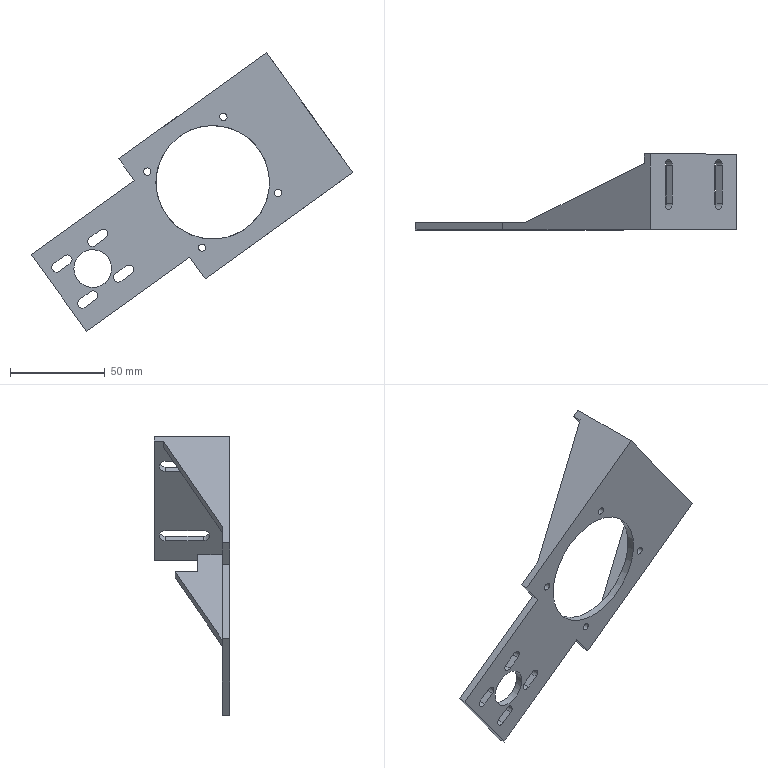Component | NX | MOTOR_MOUNTING_PLATE | 1 solid | 48 faces | volume 48278 mm3 | plane 30 | cylinder 18 | commonest cylinder face diameters 5 x8 6.6 x4 3.838 x4 60 x1 20 x1